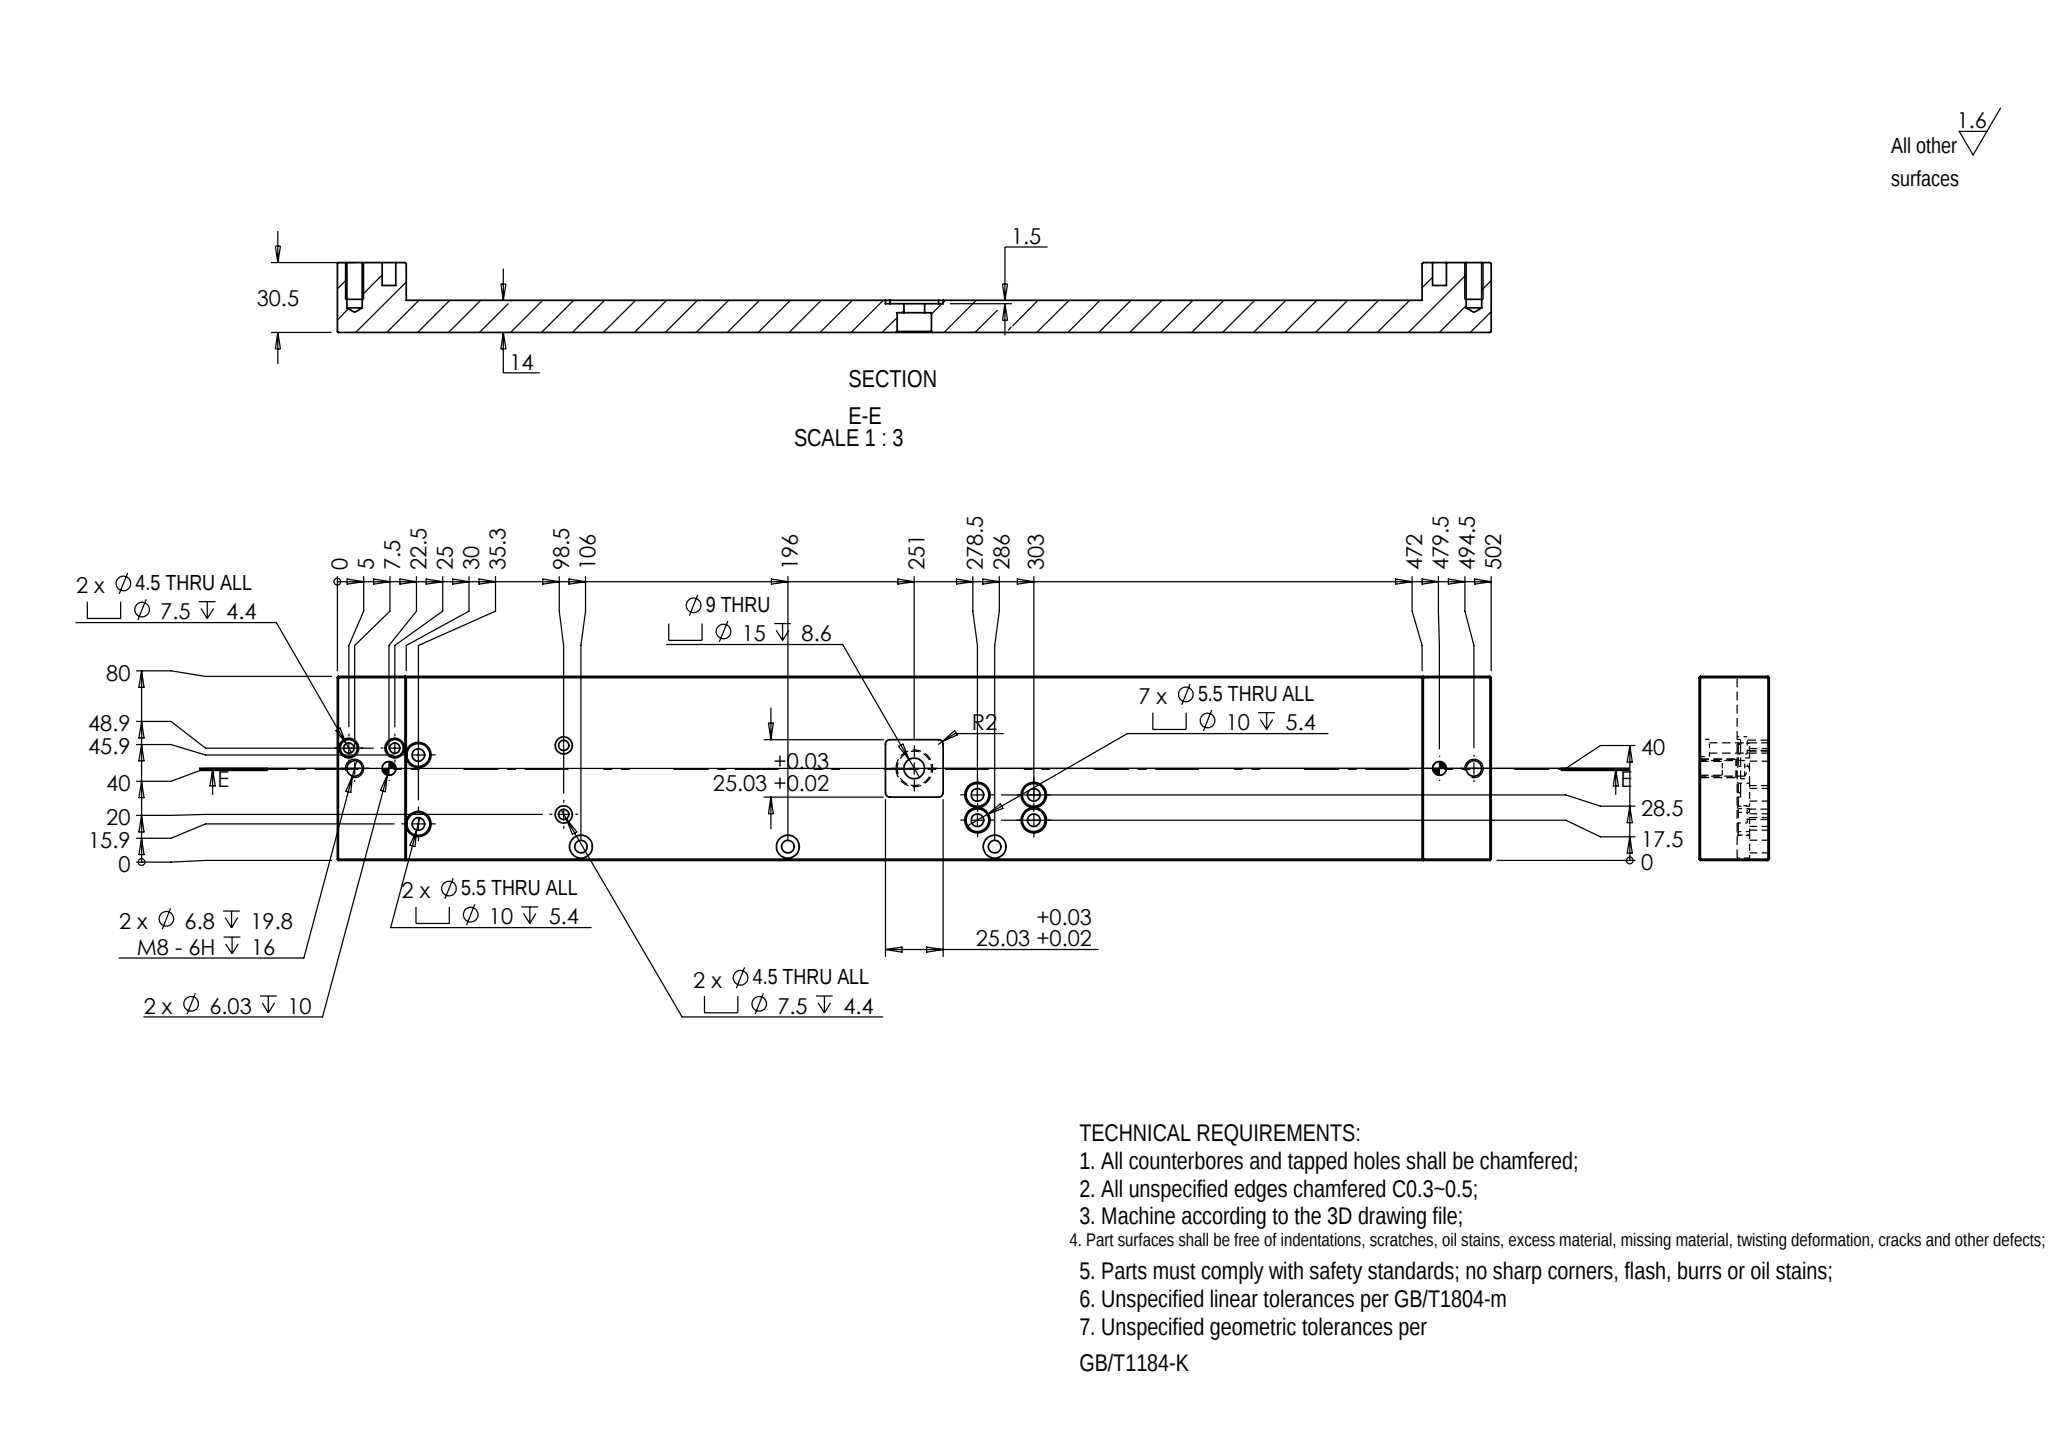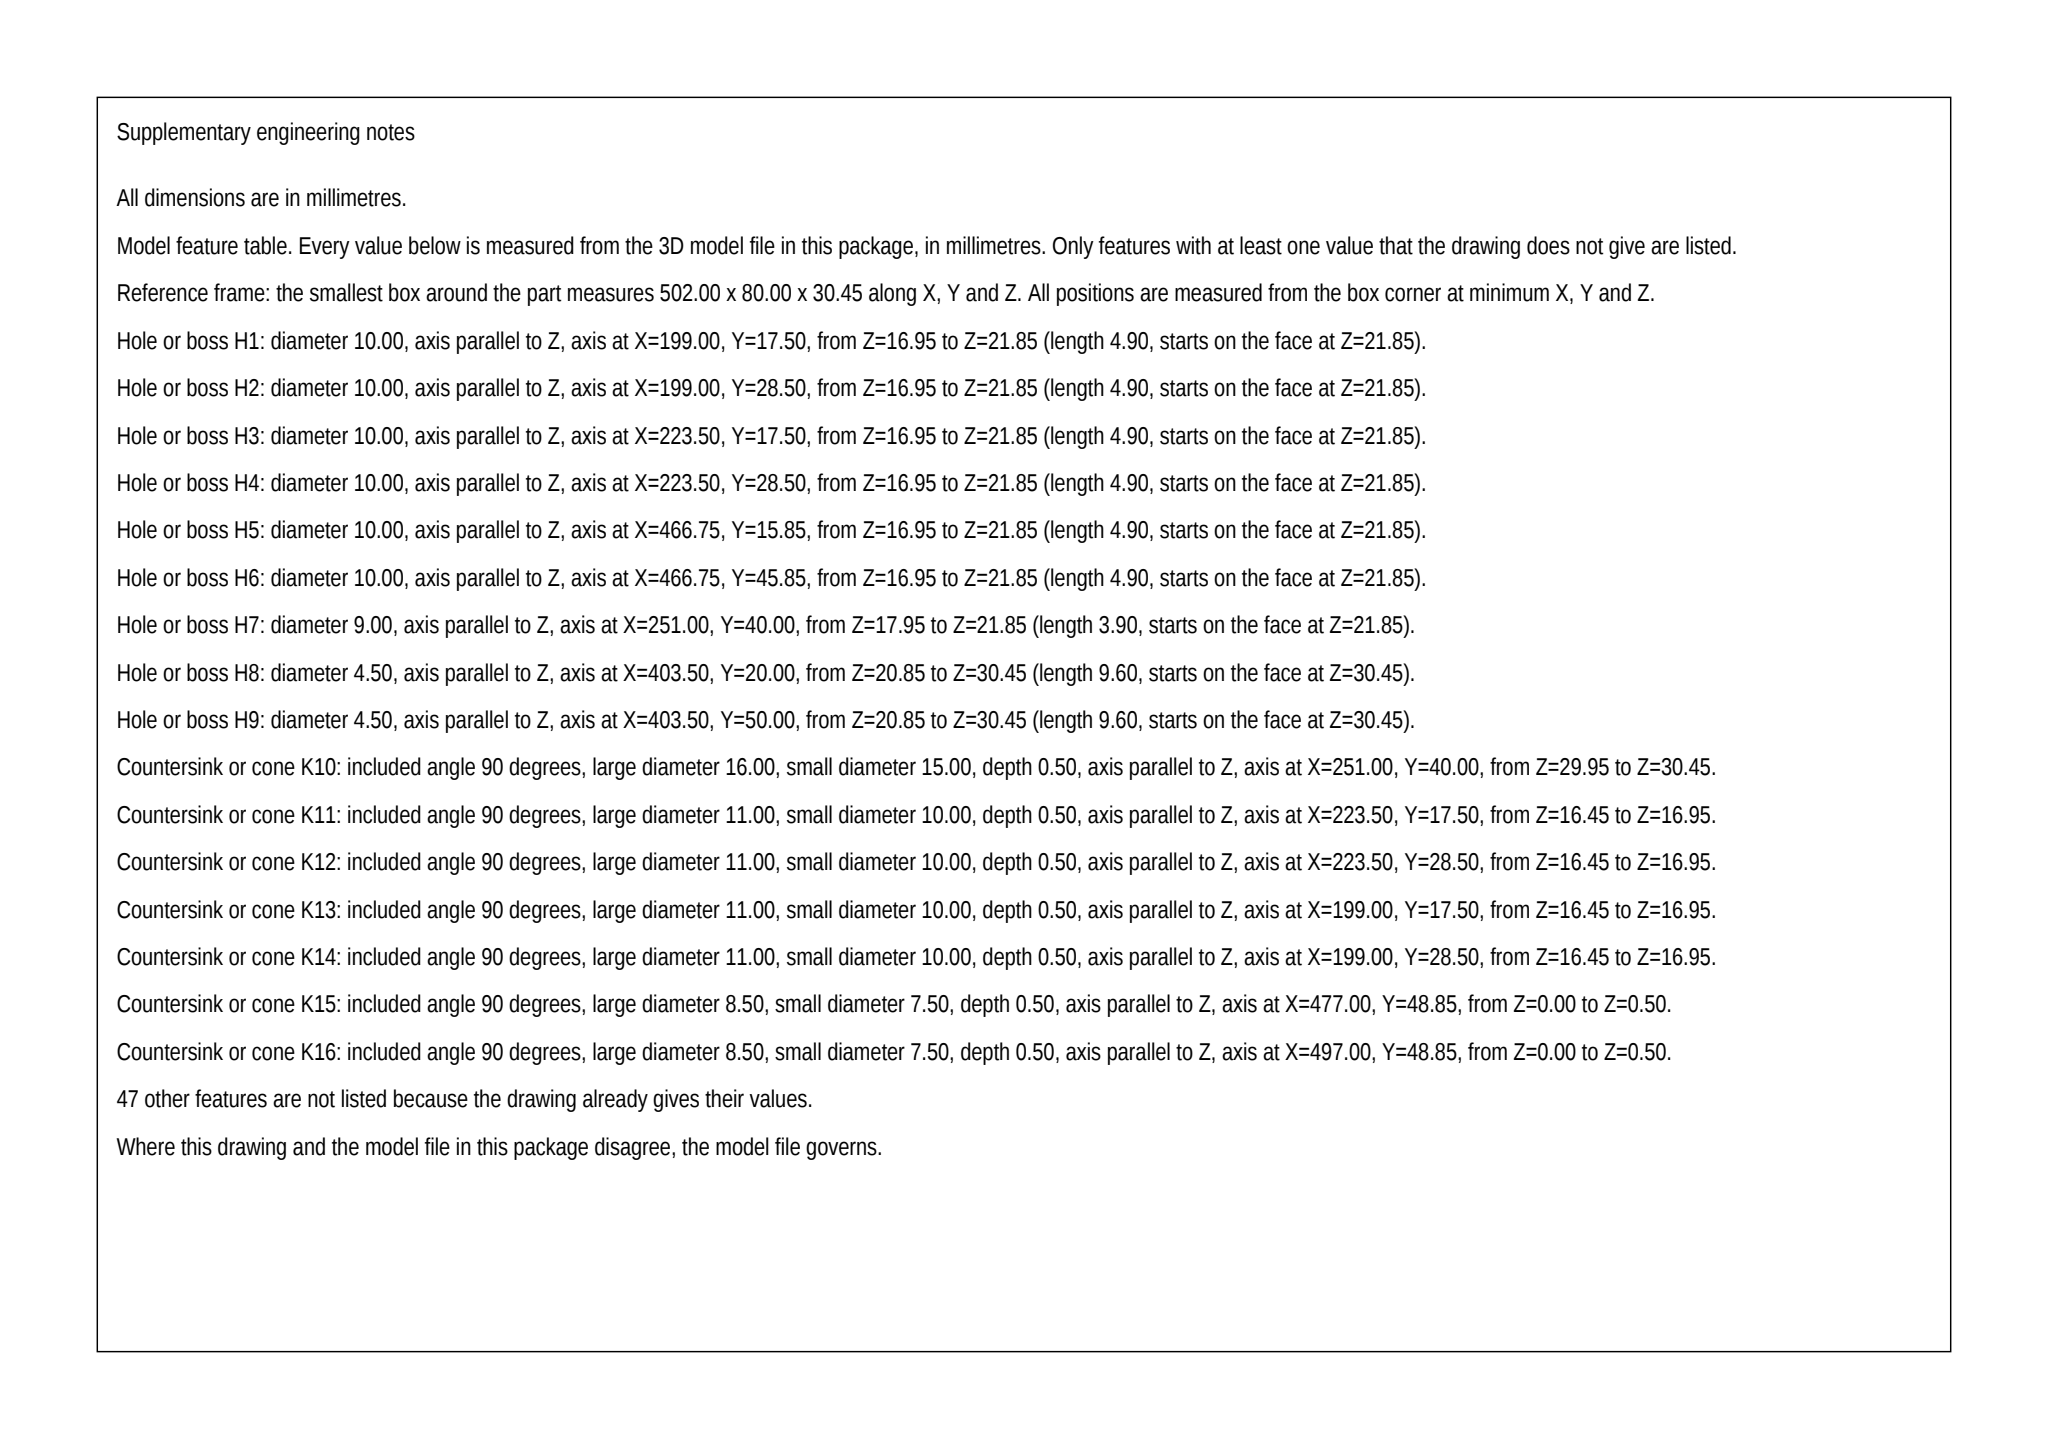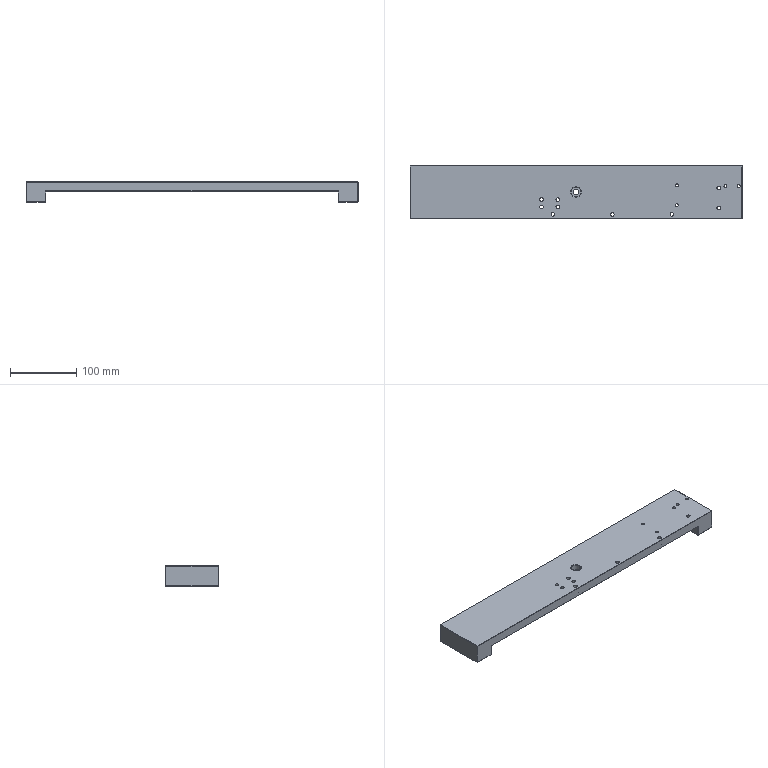Part | SolidWorks | mm | 1 solid | 155 faces | box 502 x 80 x 30.45 mm | volume 628505 mm3 | cylinder 68 | plane 65 | cone 22 | commonest cylinder face diameters 10 x18 5.5 x18 7.5 x8 4.5 x8 6.8 x4 6.03 x4 4 x4 15 x2